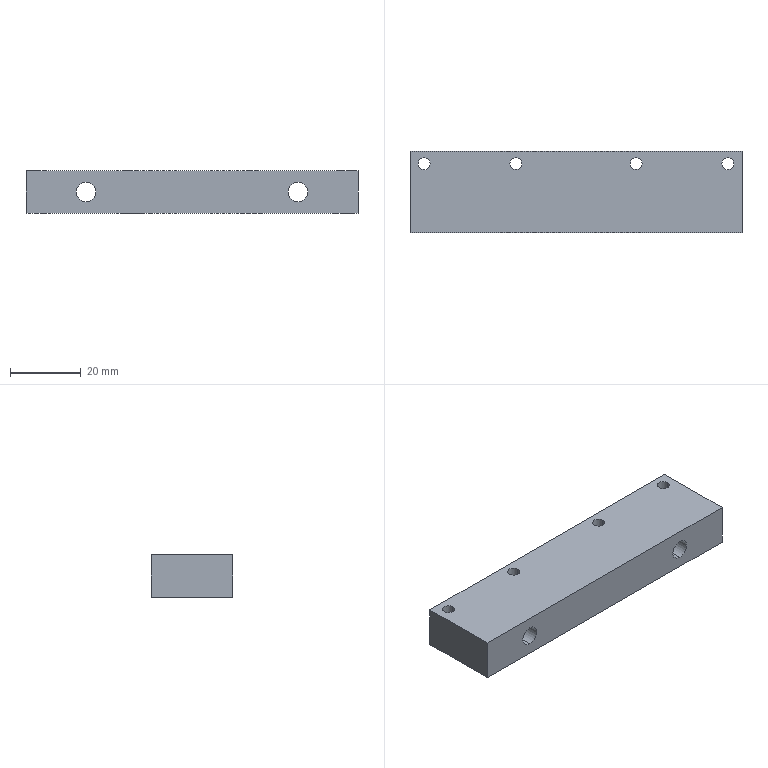Part | SolidWorks | mm | 1 solid | 36 faces | box 94 x 23 x 12 mm | volume 23563 mm3 | cylinder 24 | plane 12 | commonest cylinder face diameters 6 x8 3.4 x8 10 x4 5.5 x4
STEP:
#1=CARTESIAN_POINT('',(46.,8.,3.4));
#2=VERTEX_POINT('',#1);
#3=CARTESIAN_POINT('',(40.,8.,3.4));
#4=VERTEX_POINT('',#3);
#5=CARTESIAN_POINT('',(43.,8.,3.4));
#6=DIRECTION('',(0.,0.,-1.));
#7=DIRECTION('',(-1.,0.,0.));
#8=AXIS2_PLACEMENT_3D('',#5,#6,#7);
#9=CIRCLE('',#8,3.);
#10=EDGE_CURVE('',#2,#4,#9,.T.);
#11=ORIENTED_EDGE('',*,*,#10,.F.);
#12=CARTESIAN_POINT('',(46.,8.,0.));
#13=VERTEX_POINT('',#12);
#14=CARTESIAN_POINT('',(46.,8.,0.));
#15=DIRECTION('',(0.,0.,-1.));
#16=VECTOR('',#15,1000.);
#17=LINE('',#14,#16);
#18=EDGE_CURVE('',#2,#13,#17,.T.);
#19=ORIENTED_EDGE('',*,*,#18,.T.);
#20=CARTESIAN_POINT('',(40.,8.,0.));
#21=VERTEX_POINT('',#20);
#22=CARTESIAN_POINT('',(43.,8.,0.));
#23=DIRECTION('',(0.,0.,-1.));
#24=DIRECTION('',(-1.,0.,0.));
#25=AXIS2_PLACEMENT_3D('',#22,#23,#24);
#26=CIRCLE('',#25,3.);
#27=EDGE_CURVE('',#13,#21,#26,.T.);
#28=ORIENTED_EDGE('',*,*,#27,.T.);
#29=CARTESIAN_POINT('',(40.,8.,0.));
#30=DIRECTION('',(0.,0.,-1.));
#31=VECTOR('',#30,1000.);
#32=LINE('',#29,#31);
#33=EDGE_CURVE('',#4,#21,#32,.T.);
#34=ORIENTED_EDGE('',*,*,#33,.F.);
#35=EDGE_LOOP('',(#11,#19,#28,#34));
#36=FACE_OUTER_BOUND('',#35,.T.);
#37=CARTESIAN_POINT('',(43.,8.,0.));
#38=DIRECTION('',(0.,0.,-1.));
#39=DIRECTION('',(-1.,0.,0.));
#40=AXIS2_PLACEMENT_3D('',#37,#38,#39);
#41=CYLINDRICAL_SURFACE('',#40,3.);
#42=ADVANCED_FACE('',(#36),#41,.F.);
#43=CARTESIAN_POINT('',(44.7,8.,12.));
#44=VERTEX_POINT('',#43);
#45=CARTESIAN_POINT('',(41.3,8.,12.));
#46=VERTEX_POINT('',#45);
#47=CARTESIAN_POINT('',(43.,8.,12.));
#48=DIRECTION('',(0.,0.,-1.));
#49=DIRECTION('',(-1.,0.,0.));
#50=AXIS2_PLACEMENT_3D('',#47,#48,#49);
#51=CIRCLE('',#50,1.7);
#52=EDGE_CURVE('',#44,#46,#51,.T.);
#53=ORIENTED_EDGE('',*,*,#52,.F.);
#54=CARTESIAN_POINT('',(44.7,8.,3.4));
#55=VERTEX_POINT('',#54);
#56=CARTESIAN_POINT('',(44.7,8.,0.));
#57=DIRECTION('',(0.,0.,-1.));
#58=VECTOR('',#57,1000.);
#59=LINE('',#56,#58);
#60=EDGE_CURVE('',#44,#55,#59,.T.);
#61=ORIENTED_EDGE('',*,*,#60,.T.);
#62=CARTESIAN_POINT('',(41.3,8.,3.4));
#63=VERTEX_POINT('',#62);
#64=CARTESIAN_POINT('',(43.,8.,3.4));
#65=DIRECTION('',(0.,0.,-1.));
#66=DIRECTION('',(-1.,0.,0.));
#67=AXIS2_PLACEMENT_3D('',#64,#65,#66);
#68=CIRCLE('',#67,1.7);
#69=EDGE_CURVE('',#55,#63,#68,.T.);
#70=ORIENTED_EDGE('',*,*,#69,.T.);
#71=CARTESIAN_POINT('',(41.3,8.,0.));
#72=DIRECTION('',(0.,0.,-1.));
#73=VECTOR('',#72,1000.);
#74=LINE('',#71,#73);
#75=EDGE_CURVE('',#46,#63,#74,.T.);
#76=ORIENTED_EDGE('',*,*,#75,.F.);
#77=EDGE_LOOP('',(#53,#61,#70,#76));
#78=FACE_OUTER_BOUND('',#77,.T.);
#79=CARTESIAN_POINT('',(43.,8.,0.));
#80=DIRECTION('',(0.,0.,-1.));
#81=DIRECTION('',(-1.,0.,0.));
#82=AXIS2_PLACEMENT_3D('',#79,#80,#81);
#83=CYLINDRICAL_SURFACE('',#82,1.7);
#84=ADVANCED_FACE('',(#78),#83,.F.);
#85=CARTESIAN_POINT('',(20.,8.,3.4));
#86=VERTEX_POINT('',#85);
#87=CARTESIAN_POINT('',(14.,8.,3.4));
#88=VERTEX_POINT('',#87);
#89=CARTESIAN_POINT('',(17.,8.,3.4));
#90=DIRECTION('',(0.,0.,-1.));
#91=DIRECTION('',(-1.,0.,0.));
#92=AXIS2_PLACEMENT_3D('',#89,#90,#91);
#93=CIRCLE('',#92,3.);
#94=EDGE_CURVE('',#86,#88,#93,.T.);
#95=ORIENTED_EDGE('',*,*,#94,.F.);
#96=CARTESIAN_POINT('',(20.,8.,0.));
#97=VERTEX_POINT('',#96);
#98=CARTESIAN_POINT('',(20.,8.,0.));
#99=DIRECTION('',(0.,0.,-1.));
#100=VECTOR('',#99,1000.);
#101=LINE('',#98,#100);
#102=EDGE_CURVE('',#86,#97,#101,.T.);
#103=ORIENTED_EDGE('',*,*,#102,.T.);
#104=CARTESIAN_POINT('',(14.,8.,0.));
#105=VERTEX_POINT('',#104);
#106=CARTESIAN_POINT('',(17.,8.,0.));
#107=DIRECTION('',(0.,0.,-1.));
#108=DIRECTION('',(-1.,0.,0.));
#109=AXIS2_PLACEMENT_3D('',#106,#107,#108);
#110=CIRCLE('',#109,3.);
#111=EDGE_CURVE('',#97,#105,#110,.T.);
#112=ORIENTED_EDGE('',*,*,#111,.T.);
#113=CARTESIAN_POINT('',(14.,8.,0.));
#114=DIRECTION('',(0.,0.,-1.));
#115=VECTOR('',#114,1000.);
#116=LINE('',#113,#115);
#117=EDGE_CURVE('',#88,#105,#116,.T.);
#118=ORIENTED_EDGE('',*,*,#117,.F.);
#119=EDGE_LOOP('',(#95,#103,#112,#118));
#120=FACE_OUTER_BOUND('',#119,.T.);
#121=CARTESIAN_POINT('',(17.,8.,0.));
#122=DIRECTION('',(0.,0.,-1.));
#123=DIRECTION('',(-1.,0.,0.));
#124=AXIS2_PLACEMENT_3D('',#121,#122,#123);
#125=CYLINDRICAL_SURFACE('',#124,3.);
#126=ADVANCED_FACE('',(#120),#125,.F.);
#127=CARTESIAN_POINT('',(18.7,8.,12.));
#128=VERTEX_POINT('',#127);
#129=CARTESIAN_POINT('',(15.3,8.,12.));
#130=VERTEX_POINT('',#129);
#131=CARTESIAN_POINT('',(17.,8.,12.));
#132=DIRECTION('',(0.,0.,-1.));
#133=DIRECTION('',(-1.,0.,0.));
#134=AXIS2_PLACEMENT_3D('',#131,#132,#133);
#135=CIRCLE('',#134,1.7);
#136=EDGE_CURVE('',#128,#130,#135,.T.);
#137=ORIENTED_EDGE('',*,*,#136,.F.);
#138=CARTESIAN_POINT('',(18.7,8.,3.4));
#139=VERTEX_POINT('',#138);
#140=CARTESIAN_POINT('',(18.7,8.,0.));
#141=DIRECTION('',(0.,0.,-1.));
#142=VECTOR('',#141,1000.);
#143=LINE('',#140,#142);
#144=EDGE_CURVE('',#128,#139,#143,.T.);
#145=ORIENTED_EDGE('',*,*,#144,.T.);
#146=CARTESIAN_POINT('',(15.3,8.,3.4));
#147=VERTEX_POINT('',#146);
#148=CARTESIAN_POINT('',(17.,8.,3.4));
#149=DIRECTION('',(0.,0.,-1.));
#150=DIRECTION('',(-1.,0.,0.));
#151=AXIS2_PLACEMENT_3D('',#148,#149,#150);
#152=CIRCLE('',#151,1.7);
#153=EDGE_CURVE('',#139,#147,#152,.T.);
#154=ORIENTED_EDGE('',*,*,#153,.T.);
#155=CARTESIAN_POINT('',(15.3,8.,0.));
#156=DIRECTION('',(0.,0.,-1.));
#157=VECTOR('',#156,1000.);
#158=LINE('',#155,#157);
#159=EDGE_CURVE('',#130,#147,#158,.T.);
#160=ORIENTED_EDGE('',*,*,#159,.F.);
#161=EDGE_LOOP('',(#137,#145,#154,#160));
#162=FACE_OUTER_BOUND('',#161,.T.);
#163=CARTESIAN_POINT('',(17.,8.,0.));
#164=DIRECTION('',(0.,0.,-1.));
#165=DIRECTION('',(-1.,0.,0.));
#166=AXIS2_PLACEMENT_3D('',#163,#164,#165);
#167=CYLINDRICAL_SURFACE('',#166,1.7);
#168=ADVANCED_FACE('',(#162),#167,.F.);
#169=CARTESIAN_POINT('',(-14.,8.,3.4));
#170=VERTEX_POINT('',#169);
#171=CARTESIAN_POINT('',(-20.,8.,3.4));
#172=VERTEX_POINT('',#171);
#173=CARTESIAN_POINT('',(-17.,8.,3.4));
#174=DIRECTION('',(0.,0.,-1.));
#175=DIRECTION('',(-1.,0.,0.));
#176=AXIS2_PLACEMENT_3D('',#173,#174,#175);
#177=CIRCLE('',#176,3.);
#178=EDGE_CURVE('',#170,#172,#177,.T.);
#179=ORIENTED_EDGE('',*,*,#178,.F.);
#180=CARTESIAN_POINT('',(-14.,8.,0.));
#181=VERTEX_POINT('',#180);
#182=CARTESIAN_POINT('',(-14.,8.,0.));
#183=DIRECTION('',(0.,0.,-1.));
#184=VECTOR('',#183,1000.);
#185=LINE('',#182,#184);
#186=EDGE_CURVE('',#170,#181,#185,.T.);
#187=ORIENTED_EDGE('',*,*,#186,.T.);
#188=CARTESIAN_POINT('',(-20.,8.,0.));
#189=VERTEX_POINT('',#188);
#190=CARTESIAN_POINT('',(-17.,8.,0.));
#191=DIRECTION('',(0.,0.,-1.));
#192=DIRECTION('',(-1.,0.,0.));
#193=AXIS2_PLACEMENT_3D('',#190,#191,#192);
#194=CIRCLE('',#193,3.);
#195=EDGE_CURVE('',#181,#189,#194,.T.);
#196=ORIENTED_EDGE('',*,*,#195,.T.);
#197=CARTESIAN_POINT('',(-20.,8.,0.));
#198=DIRECTION('',(0.,0.,-1.));
#199=VECTOR('',#198,1000.);
#200=LINE('',#197,#199);
#201=EDGE_CURVE('',#172,#189,#200,.T.);
#202=ORIENTED_EDGE('',*,*,#201,.F.);
#203=EDGE_LOOP('',(#179,#187,#196,#202));
#204=FACE_OUTER_BOUND('',#203,.T.);
#205=CARTESIAN_POINT('',(-17.,8.,0.));
#206=DIRECTION('',(0.,0.,-1.));
#207=DIRECTION('',(-1.,0.,0.));
#208=AXIS2_PLACEMENT_3D('',#205,#206,#207);
#209=CYLINDRICAL_SURFACE('',#208,3.);
#210=ADVANCED_FACE('',(#204),#209,.F.);
#211=CARTESIAN_POINT('',(-15.3,8.,12.));
#212=VERTEX_POINT('',#211);
#213=CARTESIAN_POINT('',(-18.7,8.,12.));
#214=VERTEX_POINT('',#213);
#215=CARTESIAN_POINT('',(-17.,8.,12.));
#216=DIRECTION('',(0.,0.,-1.));
#217=DIRECTION('',(-1.,0.,0.));
#218=AXIS2_PLACEMENT_3D('',#215,#216,#217);
#219=CIRCLE('',#218,1.7);
#220=EDGE_CURVE('',#212,#214,#219,.T.);
#221=ORIENTED_EDGE('',*,*,#220,.F.);
#222=CARTESIAN_POINT('',(-15.3,8.,3.4));
#223=VERTEX_POINT('',#222);
#224=CARTESIAN_POINT('',(-15.3,8.,0.));
#225=DIRECTION('',(0.,0.,-1.));
#226=VECTOR('',#225,1000.);
#227=LINE('',#224,#226);
#228=EDGE_CURVE('',#212,#223,#227,.T.);
#229=ORIENTED_EDGE('',*,*,#228,.T.);
#230=CARTESIAN_POINT('',(-18.7,8.,3.4));
#231=VERTEX_POINT('',#230);
#232=CARTESIAN_POINT('',(-17.,8.,3.4));
#233=DIRECTION('',(0.,0.,-1.));
#234=DIRECTION('',(-1.,0.,0.));
#235=AXIS2_PLACEMENT_3D('',#232,#233,#234);
#236=CIRCLE('',#235,1.7);
#237=EDGE_CURVE('',#223,#231,#236,.T.);
#238=ORIENTED_EDGE('',*,*,#237,.T.);
#239=CARTESIAN_POINT('',(-18.7,8.,0.));
#240=DIRECTION('',(0.,0.,-1.));
#241=VECTOR('',#240,1000.);
#242=LINE('',#239,#241);
#243=EDGE_CURVE('',#214,#231,#242,.T.);
#244=ORIENTED_EDGE('',*,*,#243,.F.);
#245=EDGE_LOOP('',(#221,#229,#238,#244));
#246=FACE_OUTER_BOUND('',#245,.T.);
#247=CARTESIAN_POINT('',(-17.,8.,0.));
#248=DIRECTION('',(0.,0.,-1.));
#249=DIRECTION('',(-1.,0.,0.));
#250=AXIS2_PLACEMENT_3D('',#247,#248,#249);
#251=CYLINDRICAL_SURFACE('',#250,1.7);
#252=ADVANCED_FACE('',(#246),#251,.F.);
#253=CARTESIAN_POINT('',(-40.,8.,3.4));
#254=VERTEX_POINT('',#253);
#255=CARTESIAN_POINT('',(-46.,8.,3.4));
#256=VERTEX_POINT('',#255);
#257=CARTESIAN_POINT('',(-43.,8.,3.4));
#258=DIRECTION('',(0.,0.,-1.));
#259=DIRECTION('',(-1.,0.,0.));
#260=AXIS2_PLACEMENT_3D('',#257,#258,#259);
#261=CIRCLE('',#260,3.);
#262=EDGE_CURVE('',#254,#256,#261,.T.);
#263=ORIENTED_EDGE('',*,*,#262,.F.);
#264=CARTESIAN_POINT('',(-40.,8.,0.));
#265=VERTEX_POINT('',#264);
#266=CARTESIAN_POINT('',(-40.,8.,0.));
#267=DIRECTION('',(0.,0.,-1.));
#268=VECTOR('',#267,1000.);
#269=LINE('',#266,#268);
#270=EDGE_CURVE('',#254,#265,#269,.T.);
#271=ORIENTED_EDGE('',*,*,#270,.T.);
#272=CARTESIAN_POINT('',(-46.,8.,0.));
#273=VERTEX_POINT('',#272);
#274=CARTESIAN_POINT('',(-43.,8.,0.));
#275=DIRECTION('',(0.,0.,-1.));
#276=DIRECTION('',(-1.,0.,0.));
#277=AXIS2_PLACEMENT_3D('',#274,#275,#276);
#278=CIRCLE('',#277,3.);
#279=EDGE_CURVE('',#265,#273,#278,.T.);
#280=ORIENTED_EDGE('',*,*,#279,.T.);
#281=CARTESIAN_POINT('',(-46.,8.,0.));
#282=DIRECTION('',(0.,0.,-1.));
#283=VECTOR('',#282,1000.);
#284=LINE('',#281,#283);
#285=EDGE_CURVE('',#256,#273,#284,.T.);
#286=ORIENTED_EDGE('',*,*,#285,.F.);
#287=EDGE_LOOP('',(#263,#271,#280,#286));
#288=FACE_OUTER_BOUND('',#287,.T.);
#289=CARTESIAN_POINT('',(-43.,8.,0.));
#290=DIRECTION('',(0.,0.,-1.));
#291=DIRECTION('',(-1.,0.,0.));
#292=AXIS2_PLACEMENT_3D('',#289,#290,#291);
#293=CYLINDRICAL_SURFACE('',#292,3.);
#294=ADVANCED_FACE('',(#288),#293,.F.);
#295=CARTESIAN_POINT('',(-41.3,8.,12.));
#296=VERTEX_POINT('',#295);
#297=CARTESIAN_POINT('',(-44.7,8.,12.));
#298=VERTEX_POINT('',#297);
#299=CARTESIAN_POINT('',(-43.,8.,12.));
#300=DIRECTION('',(0.,0.,-1.));
#301=DIRECTION('',(-1.,0.,0.));
#302=AXIS2_PLACEMENT_3D('',#299,#300,#301);
#303=CIRCLE('',#302,1.7);
#304=EDGE_CURVE('',#296,#298,#303,.T.);
#305=ORIENTED_EDGE('',*,*,#304,.F.);
#306=CARTESIAN_POINT('',(-41.3,8.,3.4));
#307=VERTEX_POINT('',#306);
#308=CARTESIAN_POINT('',(-41.3,8.,0.));
#309=DIRECTION('',(0.,0.,-1.));
#310=VECTOR('',#309,1000.);
#311=LINE('',#308,#310);
#312=EDGE_CURVE('',#296,#307,#311,.T.);
#313=ORIENTED_EDGE('',*,*,#312,.T.);
#314=CARTESIAN_POINT('',(-44.7,8.,3.4));
#315=VERTEX_POINT('',#314);
#316=CARTESIAN_POINT('',(-43.,8.,3.4));
#317=DIRECTION('',(0.,0.,-1.));
#318=DIRECTION('',(-1.,0.,0.));
#319=AXIS2_PLACEMENT_3D('',#316,#317,#318);
#320=CIRCLE('',#319,1.7);
#321=EDGE_CURVE('',#307,#315,#320,.T.);
#322=ORIENTED_EDGE('',*,*,#321,.T.);
#323=CARTESIAN_POINT('',(-44.7,8.,0.));
#324=DIRECTION('',(0.,0.,-1.));
#325=VECTOR('',#324,1000.);
#326=LINE('',#323,#325);
#327=EDGE_CURVE('',#298,#315,#326,.T.);
#328=ORIENTED_EDGE('',*,*,#327,.F.);
#329=EDGE_LOOP('',(#305,#313,#322,#328));
#330=FACE_OUTER_BOUND('',#329,.T.);
#331=CARTESIAN_POINT('',(-43.,8.,0.));
#332=DIRECTION('',(0.,0.,-1.));
#333=DIRECTION('',(-1.,0.,0.));
#334=AXIS2_PLACEMENT_3D('',#331,#332,#333);
#335=CYLINDRICAL_SURFACE('',#334,1.7);
#336=ADVANCED_FACE('',(#330),#335,.F.);
#337=CARTESIAN_POINT('',(-30.,6.1,1.));
#338=VERTEX_POINT('',#337);
#339=CARTESIAN_POINT('',(-30.,6.1,11.));
#340=VERTEX_POINT('',#339);
#341=CARTESIAN_POINT('',(-30.,6.1,6.));
#342=DIRECTION('',(0.,1.,0.));
#343=DIRECTION('',(0.,0.,1.));
#344=AXIS2_PLACEMENT_3D('',#341,#342,#343);
#345=CIRCLE('',#344,5.);
#346=EDGE_CURVE('',#338,#340,#345,.T.);
#347=ORIENTED_EDGE('',*,*,#346,.F.);
#348=CARTESIAN_POINT('',(-30.,11.5,1.));
#349=VERTEX_POINT('',#348);
#350=CARTESIAN_POINT('',(-30.,11.5,1.));
#351=DIRECTION('',(0.,1.,0.));
#352=VECTOR('',#351,1000.);
#353=LINE('',#350,#352);
#354=EDGE_CURVE('',#338,#349,#353,.T.);
#355=ORIENTED_EDGE('',*,*,#354,.T.);
#356=CARTESIAN_POINT('',(-30.,11.5,11.));
#357=VERTEX_POINT('',#356);
#358=CARTESIAN_POINT('',(-30.,11.5,6.));
#359=DIRECTION('',(0.,1.,0.));
#360=DIRECTION('',(0.,0.,1.));
#361=AXIS2_PLACEMENT_3D('',#358,#359,#360);
#362=CIRCLE('',#361,5.);
#363=EDGE_CURVE('',#349,#357,#362,.T.);
#364=ORIENTED_EDGE('',*,*,#363,.T.);
#365=CARTESIAN_POINT('',(-30.,11.5,11.));
#366=DIRECTION('',(0.,1.,0.));
#367=VECTOR('',#366,1000.);
#368=LINE('',#365,#367);
#369=EDGE_CURVE('',#340,#357,#368,.T.);
#370=ORIENTED_EDGE('',*,*,#369,.F.);
#371=EDGE_LOOP('',(#347,#355,#364,#370));
#372=FACE_OUTER_BOUND('',#371,.T.);
#373=CARTESIAN_POINT('',(-30.,11.5,6.));
#374=DIRECTION('',(0.,1.,0.));
#375=DIRECTION('',(0.,0.,1.));
#376=AXIS2_PLACEMENT_3D('',#373,#374,#375);
#377=CYLINDRICAL_SURFACE('',#376,5.);
#378=ADVANCED_FACE('',(#372),#377,.F.);
#379=CARTESIAN_POINT('',(-30.,-11.5,3.25));
#380=VERTEX_POINT('',#379);
#381=CARTESIAN_POINT('',(-30.,-11.5,8.75));
#382=VERTEX_POINT('',#381);
#383=CARTESIAN_POINT('',(-30.,-11.5,6.));
#384=DIRECTION('',(0.,1.,0.));
#385=DIRECTION('',(0.,0.,1.));
#386=AXIS2_PLACEMENT_3D('',#383,#384,#385);
#387=CIRCLE('',#386,2.75);
#388=EDGE_CURVE('',#380,#382,#387,.T.);
#389=ORIENTED_EDGE('',*,*,#388,.F.);
#390=CARTESIAN_POINT('',(-30.,6.1,3.25));
#391=VERTEX_POINT('',#390);
#392=CARTESIAN_POINT('',(-30.,11.5,3.25));
#393=DIRECTION('',(0.,1.,0.));
#394=VECTOR('',#393,1000.);
#395=LINE('',#392,#394);
#396=EDGE_CURVE('',#380,#391,#395,.T.);
#397=ORIENTED_EDGE('',*,*,#396,.T.);
#398=CARTESIAN_POINT('',(-30.,6.1,8.75));
#399=VERTEX_POINT('',#398);
#400=CARTESIAN_POINT('',(-30.,6.1,6.));
#401=DIRECTION('',(0.,1.,0.));
#402=DIRECTION('',(0.,0.,1.));
#403=AXIS2_PLACEMENT_3D('',#400,#401,#402);
#404=CIRCLE('',#403,2.75);
#405=EDGE_CURVE('',#391,#399,#404,.T.);
#406=ORIENTED_EDGE('',*,*,#405,.T.);
#407=CARTESIAN_POINT('',(-30.,11.5,8.75));
#408=DIRECTION('',(0.,1.,0.));
#409=VECTOR('',#408,1000.);
#410=LINE('',#407,#409);
#411=EDGE_CURVE('',#382,#399,#410,.T.);
#412=ORIENTED_EDGE('',*,*,#411,.F.);
#413=EDGE_LOOP('',(#389,#397,#406,#412));
#414=FACE_OUTER_BOUND('',#413,.T.);
#415=CARTESIAN_POINT('',(-30.,11.5,6.));
#416=DIRECTION('',(0.,1.,0.));
#417=DIRECTION('',(0.,0.,1.));
#418=AXIS2_PLACEMENT_3D('',#415,#416,#417);
#419=CYLINDRICAL_SURFACE('',#418,2.75);
#420=ADVANCED_FACE('',(#414),#419,.F.);
#421=CARTESIAN_POINT('',(30.,6.1,1.));
#422=VERTEX_POINT('',#421);
#423=CARTESIAN_POINT('',(30.,6.1,11.));
#424=VERTEX_POINT('',#423);
#425=CARTESIAN_POINT('',(30.,6.1,6.));
#426=DIRECTION('',(0.,1.,0.));
#427=DIRECTION('',(0.,0.,1.));
#428=AXIS2_PLACEMENT_3D('',#425,#426,#427);
#429=CIRCLE('',#428,5.);
#430=EDGE_CURVE('',#422,#424,#429,.T.);
#431=ORIENTED_EDGE('',*,*,#430,.F.);
#432=CARTESIAN_POINT('',(30.,11.5,1.));
#433=VERTEX_POINT('',#432);
#434=CARTESIAN_POINT('',(30.,11.5,1.));
#435=DIRECTION('',(0.,1.,0.));
#436=VECTOR('',#435,1000.);
#437=LINE('',#434,#436);
#438=EDGE_CURVE('',#422,#433,#437,.T.);
#439=ORIENTED_EDGE('',*,*,#438,.T.);
#440=CARTESIAN_POINT('',(30.,11.5,11.));
#441=VERTEX_POINT('',#440);
#442=CARTESIAN_POINT('',(30.,11.5,6.));
#443=DIRECTION('',(0.,1.,0.));
#444=DIRECTION('',(0.,0.,1.));
#445=AXIS2_PLACEMENT_3D('',#442,#443,#444);
#446=CIRCLE('',#445,5.);
#447=EDGE_CURVE('',#433,#441,#446,.T.);
#448=ORIENTED_EDGE('',*,*,#447,.T.);
#449=CARTESIAN_POINT('',(30.,11.5,11.));
#450=DIRECTION('',(0.,1.,0.));
#451=VECTOR('',#450,1000.);
#452=LINE('',#449,#451);
#453=EDGE_CURVE('',#424,#441,#452,.T.);
#454=ORIENTED_EDGE('',*,*,#453,.F.);
#455=EDGE_LOOP('',(#431,#439,#448,#454));
#456=FACE_OUTER_BOUND('',#455,.T.);
#457=CARTESIAN_POINT('',(30.,11.5,6.));
#458=DIRECTION('',(0.,1.,0.));
#459=DIRECTION('',(0.,0.,1.));
#460=AXIS2_PLACEMENT_3D('',#457,#458,#459);
#461=CYLINDRICAL_SURFACE('',#460,5.);
#462=ADVANCED_FACE('',(#456),#461,.F.);
#463=CARTESIAN_POINT('',(30.,-11.5,3.25));
#464=VERTEX_POINT('',#463);
#465=CARTESIAN_POINT('',(30.,-11.5,8.75));
#466=VERTEX_POINT('',#465);
#467=CARTESIAN_POINT('',(30.,-11.5,6.));
#468=DIRECTION('',(0.,1.,0.));
#469=DIRECTION('',(0.,0.,1.));
#470=AXIS2_PLACEMENT_3D('',#467,#468,#469);
#471=CIRCLE('',#470,2.75);
#472=EDGE_CURVE('',#464,#466,#471,.T.);
#473=ORIENTED_EDGE('',*,*,#472,.F.);
#474=CARTESIAN_POINT('',(30.,6.1,3.25));
#475=VERTEX_POINT('',#474);
#476=CARTESIAN_POINT('',(30.,11.5,3.25));
#477=DIRECTION('',(0.,1.,0.));
#478=VECTOR('',#477,1000.);
#479=LINE('',#476,#478);
#480=EDGE_CURVE('',#464,#475,#479,.T.);
#481=ORIENTED_EDGE('',*,*,#480,.T.);
#482=CARTESIAN_POINT('',(30.,6.1,8.75));
#483=VERTEX_POINT('',#482);
#484=CARTESIAN_POINT('',(30.,6.1,6.));
#485=DIRECTION('',(0.,1.,0.));
#486=DIRECTION('',(0.,0.,1.));
#487=AXIS2_PLACEMENT_3D('',#484,#485,#486);
#488=CIRCLE('',#487,2.75);
#489=EDGE_CURVE('',#475,#483,#488,.T.);
#490=ORIENTED_EDGE('',*,*,#489,.T.);
#491=CARTESIAN_POINT('',(30.,11.5,8.75));
#492=DIRECTION('',(0.,1.,0.));
#493=VECTOR('',#492,1000.);
#494=LINE('',#491,#493);
#495=EDGE_CURVE('',#466,#483,#494,.T.);
#496=ORIENTED_EDGE('',*,*,#495,.F.);
#497=EDGE_LOOP('',(#473,#481,#490,#496));
#498=FACE_OUTER_BOUND('',#497,.T.);
#499=CARTESIAN_POINT('',(30.,11.5,6.));
#500=DIRECTION('',(0.,1.,0.));
#501=DIRECTION('',(0.,0.,1.));
#502=AXIS2_PLACEMENT_3D('',#499,#500,#501);
#503=CYLINDRICAL_SURFACE('',#502,2.75);
#504=ADVANCED_FACE('',(#498),#503,.F.);
#505=CARTESIAN_POINT('',(17.,8.,0.));
#506=DIRECTION('',(0.,0.,-1.));
#507=DIRECTION('',(-1.,0.,0.));
#508=AXIS2_PLACEMENT_3D('',#505,#506,#507);
#509=CIRCLE('',#508,3.);
#510=EDGE_CURVE('',#105,#97,#509,.T.);
#511=ORIENTED_EDGE('',*,*,#510,.F.);
#512=ORIENTED_EDGE('',*,*,#111,.F.);
#513=EDGE_LOOP('',(#511,#512));
#514=FACE_BOUND('',#513,.T.);
#515=CARTESIAN_POINT('',(-17.,8.,0.));
#516=DIRECTION('',(0.,0.,-1.));
#517=DIRECTION('',(-1.,0.,0.));
#518=AXIS2_PLACEMENT_3D('',#515,#516,#517);
#519=CIRCLE('',#518,3.);
#520=EDGE_CURVE('',#189,#181,#519,.T.);
#521=ORIENTED_EDGE('',*,*,#520,.F.);
#522=ORIENTED_EDGE('',*,*,#195,.F.);
#523=EDGE_LOOP('',(#521,#522));
#524=FACE_BOUND('',#523,.T.);
#525=CARTESIAN_POINT('',(47.,-11.5,0.));
#526=VERTEX_POINT('',#525);
#527=CARTESIAN_POINT('',(47.,11.5,0.));
#528=VERTEX_POINT('',#527);
#529=CARTESIAN_POINT('',(47.,11.5,0.));
#530=DIRECTION('',(0.,1.,0.));
#531=VECTOR('',#530,1000.);
#532=LINE('',#529,#531);
#533=EDGE_CURVE('',#526,#528,#532,.T.);
#534=ORIENTED_EDGE('',*,*,#533,.F.);
#535=CARTESIAN_POINT('',(-47.,-11.5,0.));
#536=VERTEX_POINT('',#535);
#537=CARTESIAN_POINT('',(-47.,-11.5,0.));
#538=DIRECTION('',(1.,0.,0.));
#539=VECTOR('',#538,1000.);
#540=LINE('',#537,#539);
#541=EDGE_CURVE('',#536,#526,#540,.T.);
#542=ORIENTED_EDGE('',*,*,#541,.F.);
#543=CARTESIAN_POINT('',(-47.,11.5,0.));
#544=VERTEX_POINT('',#543);
#545=CARTESIAN_POINT('',(-47.,11.5,0.));
#546=DIRECTION('',(0.,-1.,0.));
#547=VECTOR('',#546,1000.);
#548=LINE('',#545,#547);
#549=EDGE_CURVE('',#544,#536,#548,.T.);
#550=ORIENTED_EDGE('',*,*,#549,.F.);
#551=CARTESIAN_POINT('',(-47.,11.5,0.));
#552=DIRECTION('',(-1.,0.,0.));
#553=VECTOR('',#552,1000.);
#554=LINE('',#551,#553);
#555=EDGE_CURVE('',#528,#544,#554,.T.);
#556=ORIENTED_EDGE('',*,*,#555,.F.);
#557=EDGE_LOOP('',(#534,#542,#550,#556));
#558=FACE_OUTER_BOUND('',#557,.T.);
#559=CARTESIAN_POINT('',(-43.,8.,0.));
#560=DIRECTION('',(0.,0.,-1.));
#561=DIRECTION('',(-1.,0.,0.));
#562=AXIS2_PLACEMENT_3D('',#559,#560,#561);
#563=CIRCLE('',#562,3.);
#564=EDGE_CURVE('',#273,#265,#563,.T.);
#565=ORIENTED_EDGE('',*,*,#564,.F.);
#566=ORIENTED_EDGE('',*,*,#279,.F.);
#567=EDGE_LOOP('',(#565,#566));
#568=FACE_BOUND('',#567,.T.);
#569=CARTESIAN_POINT('',(43.,8.,0.));
#570=DIRECTION('',(0.,0.,-1.));
#571=DIRECTION('',(-1.,0.,0.));
#572=AXIS2_PLACEMENT_3D('',#569,#570,#571);
#573=CIRCLE('',#572,3.);
#574=EDGE_CURVE('',#21,#13,#573,.T.);
#575=ORIENTED_EDGE('',*,*,#574,.F.);
#576=ORIENTED_EDGE('',*,*,#27,.F.);
#577=EDGE_LOOP('',(#575,#576));
#578=FACE_BOUND('',#577,.T.);
#579=CARTESIAN_POINT('',(0.,0.,0.));
#580=DIRECTION('',(0.,0.,1.));
#581=DIRECTION('',(1.,0.,0.));
#582=AXIS2_PLACEMENT_3D('',#579,#580,#581);
#583=PLANE('',#582);
#584=ADVANCED_FACE('',(#514,#524,#558,#568,#578),#583,.F.);
#585=ORIENTED_EDGE('',*,*,#533,.T.);
#586=CARTESIAN_POINT('',(47.,11.5,12.));
#587=VERTEX_POINT('',#586);
#588=CARTESIAN_POINT('',(47.,11.5,12.));
#589=DIRECTION('',(0.,0.,-1.));
#590=VECTOR('',#589,1000.);
#591=LINE('',#588,#590);
#592=EDGE_CURVE('',#587,#528,#591,.T.);
#593=ORIENTED_EDGE('',*,*,#592,.F.);
#594=CARTESIAN_POINT('',(47.,-11.5,12.));
#595=VERTEX_POINT('',#594);
#596=CARTESIAN_POINT('',(47.,11.5,12.));
#597=DIRECTION('',(0.,1.,0.));
#598=VECTOR('',#597,1000.);
#599=LINE('',#596,#598);
#600=EDGE_CURVE('',#595,#587,#599,.T.);
#601=ORIENTED_EDGE('',*,*,#600,.F.);
#602=CARTESIAN_POINT('',(47.,-11.5,12.));
#603=DIRECTION('',(0.,0.,-1.));
#604=VECTOR('',#603,1000.);
#605=LINE('',#602,#604);
#606=EDGE_CURVE('',#595,#526,#605,.T.);
#607=ORIENTED_EDGE('',*,*,#606,.T.);
#608=EDGE_LOOP('',(#585,#593,#601,#607));
#609=FACE_OUTER_BOUND('',#608,.T.);
#610=CARTESIAN_POINT('',(47.,11.5,12.));
#611=DIRECTION('',(-1.,0.,0.));
#612=DIRECTION('',(0.,0.,1.));
#613=AXIS2_PLACEMENT_3D('',#610,#611,#612);
#614=PLANE('',#613);
#615=ADVANCED_FACE('',(#609),#614,.F.);
#616=CARTESIAN_POINT('',(-30.,11.5,6.));
#617=DIRECTION('',(0.,1.,0.));
#618=DIRECTION('',(0.,0.,1.));
#619=AXIS2_PLACEMENT_3D('',#616,#617,#618);
#620=CIRCLE('',#619,5.);
#621=EDGE_CURVE('',#357,#349,#620,.T.);
#622=ORIENTED_EDGE('',*,*,#621,.F.);
#623=ORIENTED_EDGE('',*,*,#363,.F.);
#624=EDGE_LOOP('',(#622,#623));
#625=FACE_BOUND('',#624,.T.);
#626=CARTESIAN_POINT('',(30.,11.5,6.));
#627=DIRECTION('',(0.,1.,0.));
#628=DIRECTION('',(0.,0.,1.));
#629=AXIS2_PLACEMENT_3D('',#626,#627,#628);
#630=CIRCLE('',#629,5.);
#631=EDGE_CURVE('',#441,#433,#630,.T.);
#632=ORIENTED_EDGE('',*,*,#631,.F.);
#633=ORIENTED_EDGE('',*,*,#447,.F.);
#634=EDGE_LOOP('',(#632,#633));
#635=FACE_BOUND('',#634,.T.);
#636=ORIENTED_EDGE('',*,*,#555,.T.);
#637=CARTESIAN_POINT('',(-47.,11.5,12.));
#638=VERTEX_POINT('',#637);
#639=CARTESIAN_POINT('',(-47.,11.5,12.));
#640=DIRECTION('',(0.,0.,-1.));
#641=VECTOR('',#640,1000.);
#642=LINE('',#639,#641);
#643=EDGE_CURVE('',#638,#544,#642,.T.);
#644=ORIENTED_EDGE('',*,*,#643,.F.);
#645=CARTESIAN_POINT('',(-47.,11.5,12.));
#646=DIRECTION('',(-1.,0.,0.));
#647=VECTOR('',#646,1000.);
#648=LINE('',#645,#647);
#649=EDGE_CURVE('',#587,#638,#648,.T.);
#650=ORIENTED_EDGE('',*,*,#649,.F.);
#651=ORIENTED_EDGE('',*,*,#592,.T.);
#652=EDGE_LOOP('',(#636,#644,#650,#651));
#653=FACE_OUTER_BOUND('',#652,.T.);
#654=CARTESIAN_POINT('',(-47.,11.5,12.));
#655=DIRECTION('',(0.,-1.,0.));
#656=DIRECTION('',(0.,0.,-1.));
#657=AXIS2_PLACEMENT_3D('',#654,#655,#656);
#658=PLANE('',#657);
#659=ADVANCED_FACE('',(#625,#635,#653),#658,.F.);
#660=ORIENTED_EDGE('',*,*,#549,.T.);
#661=CARTESIAN_POINT('',(-47.,-11.5,12.));
#662=VERTEX_POINT('',#661);
#663=CARTESIAN_POINT('',(-47.,-11.5,12.));
#664=DIRECTION('',(0.,0.,-1.));
#665=VECTOR('',#664,1000.);
#666=LINE('',#663,#665);
#667=EDGE_CURVE('',#662,#536,#666,.T.);
#668=ORIENTED_EDGE('',*,*,#667,.F.);
#669=CARTESIAN_POINT('',(-47.,11.5,12.));
#670=DIRECTION('',(0.,-1.,0.));
#671=VECTOR('',#670,1000.);
#672=LINE('',#669,#671);
#673=EDGE_CURVE('',#638,#662,#672,.T.);
#674=ORIENTED_EDGE('',*,*,#673,.F.);
#675=ORIENTED_EDGE('',*,*,#643,.T.);
#676=EDGE_LOOP('',(#660,#668,#674,#675));
#677=FACE_OUTER_BOUND('',#676,.T.);
#678=CARTESIAN_POINT('',(-47.,11.5,12.));
#679=DIRECTION('',(1.,0.,0.));
#680=DIRECTION('',(0.,0.,-1.));
#681=AXIS2_PLACEMENT_3D('',#678,#679,#680);
#682=PLANE('',#681);
#683=ADVANCED_FACE('',(#677),#682,.F.);
#684=CARTESIAN_POINT('',(-30.,-11.5,6.));
#685=DIRECTION('',(0.,1.,0.));
#686=DIRECTION('',(0.,0.,1.));
#687=AXIS2_PLACEMENT_3D('',#684,#685,#686);
#688=CIRCLE('',#687,2.75);
#689=EDGE_CURVE('',#382,#380,#688,.T.);
#690=ORIENTED_EDGE('',*,*,#689,.T.);
#691=ORIENTED_EDGE('',*,*,#388,.T.);
#692=EDGE_LOOP('',(#690,#691));
#693=FACE_BOUND('',#692,.T.);
#694=CARTESIAN_POINT('',(30.,-11.5,6.));
#695=DIRECTION('',(0.,1.,0.));
#696=DIRECTION('',(0.,0.,1.));
#697=AXIS2_PLACEMENT_3D('',#694,#695,#696);
#698=CIRCLE('',#697,2.75);
#699=EDGE_CURVE('',#466,#464,#698,.T.);
#700=ORIENTED_EDGE('',*,*,#699,.T.);
#701=ORIENTED_EDGE('',*,*,#472,.T.);
#702=EDGE_LOOP('',(#700,#701));
#703=FACE_BOUND('',#702,.T.);
#704=ORIENTED_EDGE('',*,*,#541,.T.);
#705=ORIENTED_EDGE('',*,*,#606,.F.);
#706=CARTESIAN_POINT('',(-47.,-11.5,12.));
#707=DIRECTION('',(1.,0.,0.));
#708=VECTOR('',#707,1000.);
#709=LINE('',#706,#708);
#710=EDGE_CURVE('',#662,#595,#709,.T.);
#711=ORIENTED_EDGE('',*,*,#710,.F.);
#712=ORIENTED_EDGE('',*,*,#667,.T.);
#713=EDGE_LOOP('',(#704,#705,#711,#712));
#714=FACE_OUTER_BOUND('',#713,.T.);
#715=CARTESIAN_POINT('',(-47.,-11.5,12.));
#716=DIRECTION('',(0.,1.,0.));
#717=DIRECTION('',(0.,0.,1.));
#718=AXIS2_PLACEMENT_3D('',#715,#716,#717);
#719=PLANE('',#718);
#720=ADVANCED_FACE('',(#693,#703,#714),#719,.F.);
#721=CARTESIAN_POINT('',(43.,8.,12.));
#722=DIRECTION('',(0.,0.,-1.));
#723=DIRECTION('',(-1.,0.,0.));
#724=AXIS2_PLACEMENT_3D('',#721,#722,#723);
#725=CIRCLE('',#724,1.7);
#726=EDGE_CURVE('',#46,#44,#725,.T.);
#727=ORIENTED_EDGE('',*,*,#726,.T.);
#728=ORIENTED_EDGE('',*,*,#52,.T.);
#729=EDGE_LOOP('',(#727,#728));
#730=FACE_BOUND('',#729,.T.);
#731=CARTESIAN_POINT('',(17.,8.,12.));
#732=DIRECTION('',(0.,0.,-1.));
#733=DIRECTION('',(-1.,0.,0.));
#734=AXIS2_PLACEMENT_3D('',#731,#732,#733);
#735=CIRCLE('',#734,1.7);
#736=EDGE_CURVE('',#130,#128,#735,.T.);
#737=ORIENTED_EDGE('',*,*,#736,.T.);
#738=ORIENTED_EDGE('',*,*,#136,.T.);
#739=EDGE_LOOP('',(#737,#738));
#740=FACE_BOUND('',#739,.T.);
#741=CARTESIAN_POINT('',(-17.,8.,12.));
#742=DIRECTION('',(0.,0.,-1.));
#743=DIRECTION('',(-1.,0.,0.));
#744=AXIS2_PLACEMENT_3D('',#741,#742,#743);
#745=CIRCLE('',#744,1.7);
#746=EDGE_CURVE('',#214,#212,#745,.T.);
#747=ORIENTED_EDGE('',*,*,#746,.T.);
#748=ORIENTED_EDGE('',*,*,#220,.T.);
#749=EDGE_LOOP('',(#747,#748));
#750=FACE_BOUND('',#749,.T.);
#751=CARTESIAN_POINT('',(-43.,8.,12.));
#752=DIRECTION('',(0.,0.,-1.));
#753=DIRECTION('',(-1.,0.,0.));
#754=AXIS2_PLACEMENT_3D('',#751,#752,#753);
#755=CIRCLE('',#754,1.7);
#756=EDGE_CURVE('',#298,#296,#755,.T.);
#757=ORIENTED_EDGE('',*,*,#756,.T.);
#758=ORIENTED_EDGE('',*,*,#304,.T.);
#759=EDGE_LOOP('',(#757,#758));
#760=FACE_BOUND('',#759,.T.);
#761=ORIENTED_EDGE('',*,*,#600,.T.);
#762=ORIENTED_EDGE('',*,*,#649,.T.);
#763=ORIENTED_EDGE('',*,*,#673,.T.);
#764=ORIENTED_EDGE('',*,*,#710,.T.);
#765=EDGE_LOOP('',(#761,#762,#763,#764));
#766=FACE_OUTER_BOUND('',#765,.T.);
#767=CARTESIAN_POINT('',(0.,0.,12.));
#768=DIRECTION('',(0.,0.,1.));
#769=DIRECTION('',(1.,0.,0.));
#770=AXIS2_PLACEMENT_3D('',#767,#768,#769);
#771=PLANE('',#770);
#772=ADVANCED_FACE('',(#730,#740,#750,#760,#766),#771,.T.);
#773=ORIENTED_EDGE('',*,*,#480,.F.);
#774=ORIENTED_EDGE('',*,*,#699,.F.);
#775=ORIENTED_EDGE('',*,*,#495,.T.);
#776=CARTESIAN_POINT('',(30.,6.1,6.));
#777=DIRECTION('',(0.,1.,0.));
#778=DIRECTION('',(0.,0.,1.));
#779=AXIS2_PLACEMENT_3D('',#776,#777,#778);
#780=CIRCLE('',#779,2.75);
#781=EDGE_CURVE('',#483,#475,#780,.T.);
#782=ORIENTED_EDGE('',*,*,#781,.T.);
#783=EDGE_LOOP('',(#773,#774,#775,#782));
#784=FACE_OUTER_BOUND('',#783,.T.);
#785=CARTESIAN_POINT('',(30.,11.5,6.));
#786=DIRECTION('',(0.,1.,0.));
#787=DIRECTION('',(0.,0.,1.));
#788=AXIS2_PLACEMENT_3D('',#785,#786,#787);
#789=CYLINDRICAL_SURFACE('',#788,2.75);
#790=ADVANCED_FACE('',(#784),#789,.F.);
#791=ORIENTED_EDGE('',*,*,#781,.F.);
#792=ORIENTED_EDGE('',*,*,#489,.F.);
#793=EDGE_LOOP('',(#791,#792));
#794=FACE_BOUND('',#793,.T.);
#795=CARTESIAN_POINT('',(30.,6.1,6.));
#796=DIRECTION('',(0.,1.,0.));
#797=DIRECTION('',(0.,0.,1.));
#798=AXIS2_PLACEMENT_3D('',#795,#796,#797);
#799=CIRCLE('',#798,5.);
#800=EDGE_CURVE('',#424,#422,#799,.T.);
#801=ORIENTED_EDGE('',*,*,#800,.T.);
#802=ORIENTED_EDGE('',*,*,#430,.T.);
#803=EDGE_LOOP('',(#801,#802));
#804=FACE_OUTER_BOUND('',#803,.T.);
#805=CARTESIAN_POINT('',(32.75,6.1,6.));
#806=DIRECTION('',(0.,-1.,0.));
#807=DIRECTION('',(0.,0.,-1.));
#808=AXIS2_PLACEMENT_3D('',#805,#806,#807);
#809=PLANE('',#808);
#810=ADVANCED_FACE('',(#794,#804),#809,.F.);
#811=ORIENTED_EDGE('',*,*,#438,.F.);
#812=ORIENTED_EDGE('',*,*,#800,.F.);
#813=ORIENTED_EDGE('',*,*,#453,.T.);
#814=ORIENTED_EDGE('',*,*,#631,.T.);
#815=EDGE_LOOP('',(#811,#812,#813,#814));
#816=FACE_OUTER_BOUND('',#815,.T.);
#817=CARTESIAN_POINT('',(30.,11.5,6.));
#818=DIRECTION('',(0.,1.,0.));
#819=DIRECTION('',(0.,0.,1.));
#820=AXIS2_PLACEMENT_3D('',#817,#818,#819);
#821=CYLINDRICAL_SURFACE('',#820,5.);
#822=ADVANCED_FACE('',(#816),#821,.F.);
#823=ORIENTED_EDGE('',*,*,#396,.F.);
#824=ORIENTED_EDGE('',*,*,#689,.F.);
#825=ORIENTED_EDGE('',*,*,#411,.T.);
#826=CARTESIAN_POINT('',(-30.,6.1,6.));
#827=DIRECTION('',(0.,1.,0.));
#828=DIRECTION('',(0.,0.,1.));
#829=AXIS2_PLACEMENT_3D('',#826,#827,#828);
#830=CIRCLE('',#829,2.75);
#831=EDGE_CURVE('',#399,#391,#830,.T.);
#832=ORIENTED_EDGE('',*,*,#831,.T.);
#833=EDGE_LOOP('',(#823,#824,#825,#832));
#834=FACE_OUTER_BOUND('',#833,.T.);
#835=CARTESIAN_POINT('',(-30.,11.5,6.));
#836=DIRECTION('',(0.,1.,0.));
#837=DIRECTION('',(0.,0.,1.));
#838=AXIS2_PLACEMENT_3D('',#835,#836,#837);
#839=CYLINDRICAL_SURFACE('',#838,2.75);
#840=ADVANCED_FACE('',(#834),#839,.F.);
#841=ORIENTED_EDGE('',*,*,#831,.F.);
#842=ORIENTED_EDGE('',*,*,#405,.F.);
#843=EDGE_LOOP('',(#841,#842));
#844=FACE_BOUND('',#843,.T.);
#845=CARTESIAN_POINT('',(-30.,6.1,6.));
#846=DIRECTION('',(0.,1.,0.));
#847=DIRECTION('',(0.,0.,1.));
#848=AXIS2_PLACEMENT_3D('',#845,#846,#847);
#849=CIRCLE('',#848,5.);
#850=EDGE_CURVE('',#340,#338,#849,.T.);
#851=ORIENTED_EDGE('',*,*,#850,.T.);
#852=ORIENTED_EDGE('',*,*,#346,.T.);
#853=EDGE_LOOP('',(#851,#852));
#854=FACE_OUTER_BOUND('',#853,.T.);
#855=CARTESIAN_POINT('',(-27.25,6.1,6.));
#856=DIRECTION('',(0.,-1.,0.));
#857=DIRECTION('',(0.,0.,-1.));
#858=AXIS2_PLACEMENT_3D('',#855,#856,#857);
#859=PLANE('',#858);
#860=ADVANCED_FACE('',(#844,#854),#859,.F.);
#861=ORIENTED_EDGE('',*,*,#354,.F.);
#862=ORIENTED_EDGE('',*,*,#850,.F.);
#863=ORIENTED_EDGE('',*,*,#369,.T.);
#864=ORIENTED_EDGE('',*,*,#621,.T.);
#865=EDGE_LOOP('',(#861,#862,#863,#864));
#866=FACE_OUTER_BOUND('',#865,.T.);
#867=CARTESIAN_POINT('',(-30.,11.5,6.));
#868=DIRECTION('',(0.,1.,0.));
#869=DIRECTION('',(0.,0.,1.));
#870=AXIS2_PLACEMENT_3D('',#867,#868,#869);
#871=CYLINDRICAL_SURFACE('',#870,5.);
#872=ADVANCED_FACE('',(#866),#871,.F.);
#873=ORIENTED_EDGE('',*,*,#312,.F.);
#874=ORIENTED_EDGE('',*,*,#756,.F.);
#875=ORIENTED_EDGE('',*,*,#327,.T.);
#876=CARTESIAN_POINT('',(-43.,8.,3.4));
#877=DIRECTION('',(0.,0.,-1.));
#878=DIRECTION('',(-1.,0.,0.));
#879=AXIS2_PLACEMENT_3D('',#876,#877,#878);
#880=CIRCLE('',#879,1.7);
#881=EDGE_CURVE('',#315,#307,#880,.T.);
#882=ORIENTED_EDGE('',*,*,#881,.T.);
#883=EDGE_LOOP('',(#873,#874,#875,#882));
#884=FACE_OUTER_BOUND('',#883,.T.);
#885=CARTESIAN_POINT('',(-43.,8.,0.));
#886=DIRECTION('',(0.,0.,-1.));
#887=DIRECTION('',(-1.,0.,0.));
#888=AXIS2_PLACEMENT_3D('',#885,#886,#887);
#889=CYLINDRICAL_SURFACE('',#888,1.7);
#890=ADVANCED_FACE('',(#884),#889,.F.);
#891=ORIENTED_EDGE('',*,*,#881,.F.);
#892=ORIENTED_EDGE('',*,*,#321,.F.);
#893=EDGE_LOOP('',(#891,#892));
#894=FACE_BOUND('',#893,.T.);
#895=CARTESIAN_POINT('',(-43.,8.,3.4));
#896=DIRECTION('',(0.,0.,-1.));
#897=DIRECTION('',(-1.,0.,0.));
#898=AXIS2_PLACEMENT_3D('',#895,#896,#897);
#899=CIRCLE('',#898,3.);
#900=EDGE_CURVE('',#256,#254,#899,.T.);
#901=ORIENTED_EDGE('',*,*,#900,.T.);
#902=ORIENTED_EDGE('',*,*,#262,.T.);
#903=EDGE_LOOP('',(#901,#902));
#904=FACE_OUTER_BOUND('',#903,.T.);
#905=CARTESIAN_POINT('',(-41.3,8.,3.4));
#906=DIRECTION('',(0.,0.,1.));
#907=DIRECTION('',(1.,0.,0.));
#908=AXIS2_PLACEMENT_3D('',#905,#906,#907);
#909=PLANE('',#908);
#910=ADVANCED_FACE('',(#894,#904),#909,.F.);
#911=ORIENTED_EDGE('',*,*,#270,.F.);
#912=ORIENTED_EDGE('',*,*,#900,.F.);
#913=ORIENTED_EDGE('',*,*,#285,.T.);
#914=ORIENTED_EDGE('',*,*,#564,.T.);
#915=EDGE_LOOP('',(#911,#912,#913,#914));
#916=FACE_OUTER_BOUND('',#915,.T.);
#917=CARTESIAN_POINT('',(-43.,8.,0.));
#918=DIRECTION('',(0.,0.,-1.));
#919=DIRECTION('',(-1.,0.,0.));
#920=AXIS2_PLACEMENT_3D('',#917,#918,#919);
#921=CYLINDRICAL_SURFACE('',#920,3.);
#922=ADVANCED_FACE('',(#916),#921,.F.);
#923=ORIENTED_EDGE('',*,*,#228,.F.);
#924=ORIENTED_EDGE('',*,*,#746,.F.);
#925=ORIENTED_EDGE('',*,*,#243,.T.);
#926=CARTESIAN_POINT('',(-17.,8.,3.4));
#927=DIRECTION('',(0.,0.,-1.));
#928=DIRECTION('',(-1.,0.,0.));
#929=AXIS2_PLACEMENT_3D('',#926,#927,#928);
#930=CIRCLE('',#929,1.7);
#931=EDGE_CURVE('',#231,#223,#930,.T.);
#932=ORIENTED_EDGE('',*,*,#931,.T.);
#933=EDGE_LOOP('',(#923,#924,#925,#932));
#934=FACE_OUTER_BOUND('',#933,.T.);
#935=CARTESIAN_POINT('',(-17.,8.,0.));
#936=DIRECTION('',(0.,0.,-1.));
#937=DIRECTION('',(-1.,0.,0.));
#938=AXIS2_PLACEMENT_3D('',#935,#936,#937);
#939=CYLINDRICAL_SURFACE('',#938,1.7);
#940=ADVANCED_FACE('',(#934),#939,.F.);
#941=ORIENTED_EDGE('',*,*,#931,.F.);
#942=ORIENTED_EDGE('',*,*,#237,.F.);
#943=EDGE_LOOP('',(#941,#942));
#944=FACE_BOUND('',#943,.T.);
#945=CARTESIAN_POINT('',(-17.,8.,3.4));
#946=DIRECTION('',(0.,0.,-1.));
#947=DIRECTION('',(-1.,0.,0.));
#948=AXIS2_PLACEMENT_3D('',#945,#946,#947);
#949=CIRCLE('',#948,3.);
#950=EDGE_CURVE('',#172,#170,#949,.T.);
#951=ORIENTED_EDGE('',*,*,#950,.T.);
#952=ORIENTED_EDGE('',*,*,#178,.T.);
#953=EDGE_LOOP('',(#951,#952));
#954=FACE_OUTER_BOUND('',#953,.T.);
#955=CARTESIAN_POINT('',(-15.3,8.,3.4));
#956=DIRECTION('',(0.,0.,1.));
#957=DIRECTION('',(1.,0.,0.));
#958=AXIS2_PLACEMENT_3D('',#955,#956,#957);
#959=PLANE('',#958);
#960=ADVANCED_FACE('',(#944,#954),#959,.F.);
#961=ORIENTED_EDGE('',*,*,#186,.F.);
#962=ORIENTED_EDGE('',*,*,#950,.F.);
#963=ORIENTED_EDGE('',*,*,#201,.T.);
#964=ORIENTED_EDGE('',*,*,#520,.T.);
#965=EDGE_LOOP('',(#961,#962,#963,#964));
#966=FACE_OUTER_BOUND('',#965,.T.);
#967=CARTESIAN_POINT('',(-17.,8.,0.));
#968=DIRECTION('',(0.,0.,-1.));
#969=DIRECTION('',(-1.,0.,0.));
#970=AXIS2_PLACEMENT_3D('',#967,#968,#969);
#971=CYLINDRICAL_SURFACE('',#970,3.);
#972=ADVANCED_FACE('',(#966),#971,.F.);
#973=ORIENTED_EDGE('',*,*,#144,.F.);
#974=ORIENTED_EDGE('',*,*,#736,.F.);
#975=ORIENTED_EDGE('',*,*,#159,.T.);
#976=CARTESIAN_POINT('',(17.,8.,3.4));
#977=DIRECTION('',(0.,0.,-1.));
#978=DIRECTION('',(-1.,0.,0.));
#979=AXIS2_PLACEMENT_3D('',#976,#977,#978);
#980=CIRCLE('',#979,1.7);
#981=EDGE_CURVE('',#147,#139,#980,.T.);
#982=ORIENTED_EDGE('',*,*,#981,.T.);
#983=EDGE_LOOP('',(#973,#974,#975,#982));
#984=FACE_OUTER_BOUND('',#983,.T.);
#985=CARTESIAN_POINT('',(17.,8.,0.));
#986=DIRECTION('',(0.,0.,-1.));
#987=DIRECTION('',(-1.,0.,0.));
#988=AXIS2_PLACEMENT_3D('',#985,#986,#987);
#989=CYLINDRICAL_SURFACE('',#988,1.7);
#990=ADVANCED_FACE('',(#984),#989,.F.);
#991=ORIENTED_EDGE('',*,*,#981,.F.);
#992=ORIENTED_EDGE('',*,*,#153,.F.);
#993=EDGE_LOOP('',(#991,#992));
#994=FACE_BOUND('',#993,.T.);
#995=CARTESIAN_POINT('',(17.,8.,3.4));
#996=DIRECTION('',(0.,0.,-1.));
#997=DIRECTION('',(-1.,0.,0.));
#998=AXIS2_PLACEMENT_3D('',#995,#996,#997);
#999=CIRCLE('',#998,3.);
#1000=EDGE_CURVE('',#88,#86,#999,.T.);
#1001=ORIENTED_EDGE('',*,*,#1000,.T.);
#1002=ORIENTED_EDGE('',*,*,#94,.T.);
#1003=EDGE_LOOP('',(#1001,#1002));
#1004=FACE_OUTER_BOUND('',#1003,.T.);
#1005=CARTESIAN_POINT('',(18.7,8.,3.4));
#1006=DIRECTION('',(0.,0.,1.));
#1007=DIRECTION('',(1.,0.,0.));
#1008=AXIS2_PLACEMENT_3D('',#1005,#1006,#1007);
#1009=PLANE('',#1008);
#1010=ADVANCED_FACE('',(#994,#1004),#1009,.F.);
#1011=ORIENTED_EDGE('',*,*,#102,.F.);
#1012=ORIENTED_EDGE('',*,*,#1000,.F.);
#1013=ORIENTED_EDGE('',*,*,#117,.T.);
#1014=ORIENTED_EDGE('',*,*,#510,.T.);
#1015=EDGE_LOOP('',(#1011,#1012,#1013,#1014));
#1016=FACE_OUTER_BOUND('',#1015,.T.);
#1017=CARTESIAN_POINT('',(17.,8.,0.));
#1018=DIRECTION('',(0.,0.,-1.));
#1019=DIRECTION('',(-1.,0.,0.));
#1020=AXIS2_PLACEMENT_3D('',#1017,#1018,#1019);
#1021=CYLINDRICAL_SURFACE('',#1020,3.);
#1022=ADVANCED_FACE('',(#1016),#1021,.F.);
#1023=ORIENTED_EDGE('',*,*,#60,.F.);
#1024=ORIENTED_EDGE('',*,*,#726,.F.);
#1025=ORIENTED_EDGE('',*,*,#75,.T.);
#1026=CARTESIAN_POINT('',(43.,8.,3.4));
#1027=DIRECTION('',(0.,0.,-1.));
#1028=DIRECTION('',(-1.,0.,0.));
#1029=AXIS2_PLACEMENT_3D('',#1026,#1027,#1028);
#1030=CIRCLE('',#1029,1.7);
#1031=EDGE_CURVE('',#63,#55,#1030,.T.);
#1032=ORIENTED_EDGE('',*,*,#1031,.T.);
#1033=EDGE_LOOP('',(#1023,#1024,#1025,#1032));
#1034=FACE_OUTER_BOUND('',#1033,.T.);
#1035=CARTESIAN_POINT('',(43.,8.,0.));
#1036=DIRECTION('',(0.,0.,-1.));
#1037=DIRECTION('',(-1.,0.,0.));
#1038=AXIS2_PLACEMENT_3D('',#1035,#1036,#1037);
#1039=CYLINDRICAL_SURFACE('',#1038,1.7);
#1040=ADVANCED_FACE('',(#1034),#1039,.F.);
#1041=ORIENTED_EDGE('',*,*,#1031,.F.);
#1042=ORIENTED_EDGE('',*,*,#69,.F.);
#1043=EDGE_LOOP('',(#1041,#1042));
#1044=FACE_BOUND('',#1043,.T.);
#1045=CARTESIAN_POINT('',(43.,8.,3.4));
#1046=DIRECTION('',(0.,0.,-1.));
#1047=DIRECTION('',(-1.,0.,0.));
#1048=AXIS2_PLACEMENT_3D('',#1045,#1046,#1047);
#1049=CIRCLE('',#1048,3.);
#1050=EDGE_CURVE('',#4,#2,#1049,.T.);
#1051=ORIENTED_EDGE('',*,*,#1050,.T.);
#1052=ORIENTED_EDGE('',*,*,#10,.T.);
#1053=EDGE_LOOP('',(#1051,#1052));
#1054=FACE_OUTER_BOUND('',#1053,.T.);
#1055=CARTESIAN_POINT('',(44.7,8.,3.4));
#1056=DIRECTION('',(0.,0.,1.));
#1057=DIRECTION('',(1.,0.,0.));
#1058=AXIS2_PLACEMENT_3D('',#1055,#1056,#1057);
#1059=PLANE('',#1058);
#1060=ADVANCED_FACE('',(#1044,#1054),#1059,.F.);
#1061=ORIENTED_EDGE('',*,*,#18,.F.);
#1062=ORIENTED_EDGE('',*,*,#1050,.F.);
#1063=ORIENTED_EDGE('',*,*,#33,.T.);
#1064=ORIENTED_EDGE('',*,*,#574,.T.);
#1065=EDGE_LOOP('',(#1061,#1062,#1063,#1064));
#1066=FACE_OUTER_BOUND('',#1065,.T.);
#1067=CARTESIAN_POINT('',(43.,8.,0.));
#1068=DIRECTION('',(0.,0.,-1.));
#1069=DIRECTION('',(-1.,0.,0.));
#1070=AXIS2_PLACEMENT_3D('',#1067,#1068,#1069);
#1071=CYLINDRICAL_SURFACE('',#1070,3.);
#1072=ADVANCED_FACE('',(#1066),#1071,.F.);
#1073=CLOSED_SHELL('',(#42,#84,#126,#168,#210,#252,#294,#336,#378,#420,#462,#504,#584,#615,#659,#683,#720,#772,#790,#810,#822,#840,#860,#872,#890,#910,#922,#940,#960,#972,#990,#1010,#1022,#1040,#1060,#1072));
#1074=MANIFOLD_SOLID_BREP('',#1073);
#1075=CARTESIAN_POINT('',(0.,0.,0.));
#1076=DIRECTION('',(0.,0.,1.));
#1077=DIRECTION('',(1.,0.,0.));
#1078=AXIS2_PLACEMENT_3D('',#1075,#1076,#1077);
#1079=(LENGTH_UNIT()NAMED_UNIT(*)SI_UNIT(.MILLI.,.METRE.));
#1080=UNCERTAINTY_MEASURE_WITH_UNIT(LENGTH_MEASURE(0.00001),#1079,'','');
#1081=(NAMED_UNIT(*)PLANE_ANGLE_UNIT()SI_UNIT($,.RADIAN.));
#1082=(NAMED_UNIT(*)SI_UNIT($,.STERADIAN.)SOLID_ANGLE_UNIT());
#1083=(GEOMETRIC_REPRESENTATION_CONTEXT(3)GLOBAL_UNCERTAINTY_ASSIGNED_CONTEXT((#1080))GLOBAL_UNIT_ASSIGNED_CONTEXT((#1079,#1081,#1082))REPRESENTATION_CONTEXT('',''));
#1084=ADVANCED_BREP_SHAPE_REPRESENTATION('',(#1074,#1078),#1083);